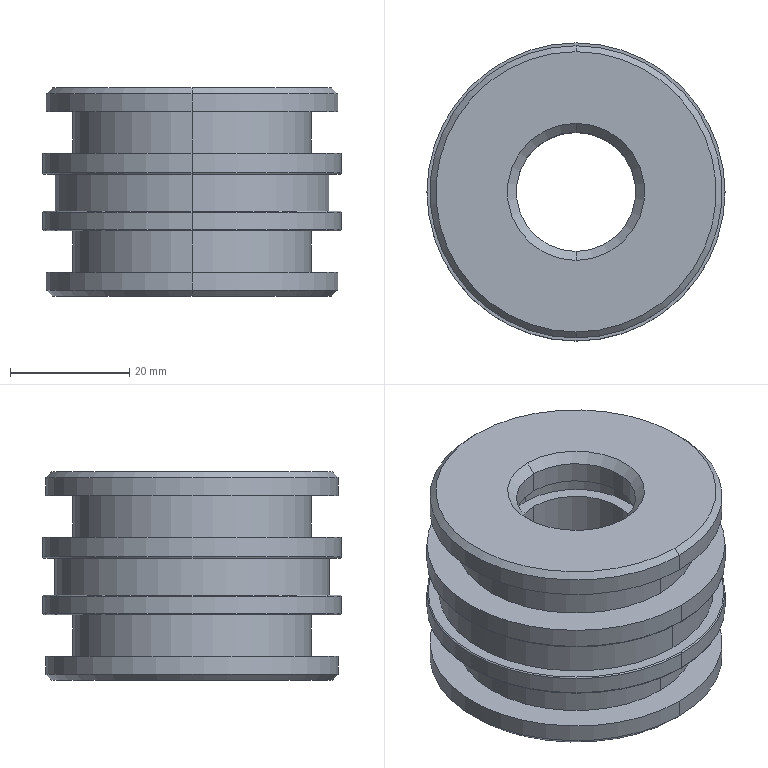Component | SolidWorks | Cylinder-1_Piston-1 | 1 solid | 42 faces | box 50 x 50 x 35 mm | volume 44660 mm3 | cylinder 20 | plane 10 | torus 6 | cone 6 | commonest cylinder face diameters 49 x4 40 x4 50 x4 20 x4 46 x2 24 x2
STEP:
#1=CARTESIAN_POINT('',(-7.109,0.06346,-12.455));
#2=VERTEX_POINT('',#1);
#3=CARTESIAN_POINT('',(-7.109,2.016,-12.455));
#4=VERTEX_POINT('',#3);
#5=CARTESIAN_POINT('',(-7.109,1.04,-12.455));
#6=DIRECTION('',(0.,-0.,-1.));
#7=DIRECTION('',(0.,1.,0.));
#8=AXIS2_PLACEMENT_3D('',#5,#6,#7);
#9=CIRCLE('',#8,0.9764);
#10=EDGE_CURVE('',#2,#4,#9,.T.);
#11=ORIENTED_EDGE('',*,*,#10,.F.);
#12=CARTESIAN_POINT('',(-7.109,0.05559,-12.447));
#13=VERTEX_POINT('',#12);
#14=CARTESIAN_POINT('',(-7.109,0.06346,-12.447));
#15=DIRECTION('',(-1.,0.,-0.));
#16=DIRECTION('',(0.,-1.,0.));
#17=AXIS2_PLACEMENT_3D('',#14,#15,#16);
#18=CIRCLE('',#17,0.007874);
#19=EDGE_CURVE('',#2,#13,#18,.T.);
#20=ORIENTED_EDGE('',*,*,#19,.T.);
#21=CARTESIAN_POINT('',(-7.109,2.024,-12.447));
#22=VERTEX_POINT('',#21);
#23=CARTESIAN_POINT('',(-7.109,1.04,-12.447));
#24=DIRECTION('',(-0.,0.,1.));
#25=DIRECTION('',(0.,1.,0.));
#26=AXIS2_PLACEMENT_3D('',#23,#24,#25);
#27=CIRCLE('',#26,0.9843);
#28=EDGE_CURVE('',#22,#13,#27,.T.);
#29=ORIENTED_EDGE('',*,*,#28,.F.);
#30=CARTESIAN_POINT('',(-7.109,2.016,-12.447));
#31=DIRECTION('',(1.,-0.,0.));
#32=DIRECTION('',(0.,1.,0.));
#33=AXIS2_PLACEMENT_3D('',#30,#31,#32);
#34=CIRCLE('',#33,0.007874);
#35=EDGE_CURVE('',#4,#22,#34,.T.);
#36=ORIENTED_EDGE('',*,*,#35,.F.);
#37=EDGE_LOOP('',(#11,#20,#29,#36));
#38=FACE_OUTER_BOUND('',#37,.T.);
#39=CARTESIAN_POINT('',(-7.109,1.04,-12.447));
#40=DIRECTION('',(-0.,0.,1.));
#41=DIRECTION('',(0.,1.,-0.));
#42=AXIS2_PLACEMENT_3D('',#39,#40,#41);
#43=TOROIDAL_SURFACE('',#42,0.9764,0.007874);
#44=ADVANCED_FACE('',(#38),#43,.T.);
#45=CARTESIAN_POINT('',(-7.109,2.016,-12.326));
#46=VERTEX_POINT('',#45);
#47=CARTESIAN_POINT('',(-7.109,0.06346,-12.326));
#48=VERTEX_POINT('',#47);
#49=CARTESIAN_POINT('',(-7.109,1.04,-12.326));
#50=DIRECTION('',(-0.,0.,1.));
#51=DIRECTION('',(0.,-1.,0.));
#52=AXIS2_PLACEMENT_3D('',#49,#50,#51);
#53=CIRCLE('',#52,0.9764);
#54=EDGE_CURVE('',#46,#48,#53,.T.);
#55=ORIENTED_EDGE('',*,*,#54,.F.);
#56=CARTESIAN_POINT('',(-7.109,2.024,-12.334));
#57=VERTEX_POINT('',#56);
#58=CARTESIAN_POINT('',(-7.109,2.016,-12.334));
#59=DIRECTION('',(-1.,-0.,-0.));
#60=DIRECTION('',(0.,-1.,0.));
#61=AXIS2_PLACEMENT_3D('',#58,#59,#60);
#62=CIRCLE('',#61,0.007874);
#63=EDGE_CURVE('',#46,#57,#62,.T.);
#64=ORIENTED_EDGE('',*,*,#63,.T.);
#65=CARTESIAN_POINT('',(-7.109,0.05559,-12.334));
#66=VERTEX_POINT('',#65);
#67=CARTESIAN_POINT('',(-7.109,1.04,-12.334));
#68=DIRECTION('',(0.,-0.,-1.));
#69=DIRECTION('',(0.,-1.,0.));
#70=AXIS2_PLACEMENT_3D('',#67,#68,#69);
#71=CIRCLE('',#70,0.9843);
#72=EDGE_CURVE('',#66,#57,#71,.T.);
#73=ORIENTED_EDGE('',*,*,#72,.F.);
#74=CARTESIAN_POINT('',(-7.109,0.06346,-12.334));
#75=DIRECTION('',(1.,-0.,0.));
#76=DIRECTION('',(0.,1.,0.));
#77=AXIS2_PLACEMENT_3D('',#74,#75,#76);
#78=CIRCLE('',#77,0.007874);
#79=EDGE_CURVE('',#48,#66,#78,.T.);
#80=ORIENTED_EDGE('',*,*,#79,.F.);
#81=EDGE_LOOP('',(#55,#64,#73,#80));
#82=FACE_OUTER_BOUND('',#81,.T.);
#83=CARTESIAN_POINT('',(-7.109,1.04,-12.334));
#84=DIRECTION('',(0.,-0.,-1.));
#85=DIRECTION('',(-0.,-1.,0.));
#86=AXIS2_PLACEMENT_3D('',#83,#84,#85);
#87=TOROIDAL_SURFACE('',#86,0.9764,0.007874);
#88=ADVANCED_FACE('',(#82),#87,.T.);
#89=CARTESIAN_POINT('',(-7.109,0.06346,-12.081));
#90=VERTEX_POINT('',#89);
#91=CARTESIAN_POINT('',(-7.109,2.016,-12.081));
#92=VERTEX_POINT('',#91);
#93=CARTESIAN_POINT('',(-7.109,1.04,-12.081));
#94=DIRECTION('',(0.,-0.,-1.));
#95=DIRECTION('',(0.,1.,0.));
#96=AXIS2_PLACEMENT_3D('',#93,#94,#95);
#97=CIRCLE('',#96,0.9764);
#98=EDGE_CURVE('',#90,#92,#97,.T.);
#99=ORIENTED_EDGE('',*,*,#98,.F.);
#100=CARTESIAN_POINT('',(-7.109,0.05559,-12.073));
#101=VERTEX_POINT('',#100);
#102=CARTESIAN_POINT('',(-7.109,0.06346,-12.073));
#103=DIRECTION('',(-1.,0.,-0.));
#104=DIRECTION('',(0.,-1.,0.));
#105=AXIS2_PLACEMENT_3D('',#102,#103,#104);
#106=CIRCLE('',#105,0.007874);
#107=EDGE_CURVE('',#90,#101,#106,.T.);
#108=ORIENTED_EDGE('',*,*,#107,.T.);
#109=CARTESIAN_POINT('',(-7.109,2.024,-12.073));
#110=VERTEX_POINT('',#109);
#111=CARTESIAN_POINT('',(-7.109,1.04,-12.073));
#112=DIRECTION('',(-0.,0.,1.));
#113=DIRECTION('',(0.,1.,0.));
#114=AXIS2_PLACEMENT_3D('',#111,#112,#113);
#115=CIRCLE('',#114,0.9843);
#116=EDGE_CURVE('',#110,#101,#115,.T.);
#117=ORIENTED_EDGE('',*,*,#116,.F.);
#118=CARTESIAN_POINT('',(-7.109,2.016,-12.073));
#119=DIRECTION('',(1.,-0.,0.));
#120=DIRECTION('',(0.,1.,0.));
#121=AXIS2_PLACEMENT_3D('',#118,#119,#120);
#122=CIRCLE('',#121,0.007874);
#123=EDGE_CURVE('',#92,#110,#122,.T.);
#124=ORIENTED_EDGE('',*,*,#123,.F.);
#125=EDGE_LOOP('',(#99,#108,#117,#124));
#126=FACE_OUTER_BOUND('',#125,.T.);
#127=CARTESIAN_POINT('',(-7.109,1.04,-12.073));
#128=DIRECTION('',(-0.,0.,1.));
#129=DIRECTION('',(0.,1.,-0.));
#130=AXIS2_PLACEMENT_3D('',#127,#128,#129);
#131=TOROIDAL_SURFACE('',#130,0.9764,0.007874);
#132=ADVANCED_FACE('',(#126),#131,.T.);
#133=CARTESIAN_POINT('',(-7.109,1.965,-11.51));
#134=VERTEX_POINT('',#133);
#135=CARTESIAN_POINT('',(-7.109,0.1146,-11.51));
#136=VERTEX_POINT('',#135);
#137=CARTESIAN_POINT('',(-7.109,1.04,-11.51));
#138=DIRECTION('',(-0.,0.,1.));
#139=DIRECTION('',(0.,-1.,0.));
#140=AXIS2_PLACEMENT_3D('',#137,#138,#139);
#141=CIRCLE('',#140,0.9252);
#142=EDGE_CURVE('',#134,#136,#141,.T.);
#143=ORIENTED_EDGE('',*,*,#142,.F.);
#144=CARTESIAN_POINT('',(-7.109,2.004,-11.549));
#145=VERTEX_POINT('',#144);
#146=CARTESIAN_POINT('',(-7.109,1.965,-11.51));
#147=DIRECTION('',(-0.,0.7071,-0.7071));
#148=VECTOR('',#147,39.37);
#149=LINE('',#146,#148);
#150=EDGE_CURVE('',#134,#145,#149,.T.);
#151=ORIENTED_EDGE('',*,*,#150,.T.);
#152=CARTESIAN_POINT('',(-7.109,0.07527,-11.549));
#153=VERTEX_POINT('',#152);
#154=CARTESIAN_POINT('',(-7.109,1.04,-11.549));
#155=DIRECTION('',(0.,-0.,-1.));
#156=DIRECTION('',(0.,-1.,0.));
#157=AXIS2_PLACEMENT_3D('',#154,#155,#156);
#158=CIRCLE('',#157,0.9646);
#159=EDGE_CURVE('',#153,#145,#158,.T.);
#160=ORIENTED_EDGE('',*,*,#159,.F.);
#161=CARTESIAN_POINT('',(-7.109,0.1146,-11.51));
#162=DIRECTION('',(-0.,-0.7071,-0.7071));
#163=VECTOR('',#162,39.37);
#164=LINE('',#161,#163);
#165=EDGE_CURVE('',#136,#153,#164,.T.);
#166=ORIENTED_EDGE('',*,*,#165,.F.);
#167=EDGE_LOOP('',(#143,#151,#160,#166));
#168=FACE_OUTER_BOUND('',#167,.T.);
#169=CARTESIAN_POINT('',(-7.109,1.04,-11.51));
#170=DIRECTION('',(0.,-0.,-1.));
#171=DIRECTION('',(0.,-1.,0.));
#172=AXIS2_PLACEMENT_3D('',#169,#170,#171);
#173=CONICAL_SURFACE('',#172,0.9252,0.7854);
#174=ADVANCED_FACE('',(#168),#173,.T.);
#175=CARTESIAN_POINT('',(-7.109,0.1146,-12.888));
#176=VERTEX_POINT('',#175);
#177=CARTESIAN_POINT('',(-7.109,1.965,-12.888));
#178=VERTEX_POINT('',#177);
#179=CARTESIAN_POINT('',(-7.109,1.04,-12.888));
#180=DIRECTION('',(0.,-0.,-1.));
#181=DIRECTION('',(0.,1.,0.));
#182=AXIS2_PLACEMENT_3D('',#179,#180,#181);
#183=CIRCLE('',#182,0.9252);
#184=EDGE_CURVE('',#176,#178,#183,.T.);
#185=ORIENTED_EDGE('',*,*,#184,.F.);
#186=CARTESIAN_POINT('',(-7.109,0.07527,-12.848));
#187=VERTEX_POINT('',#186);
#188=CARTESIAN_POINT('',(-7.109,0.07527,-12.848));
#189=DIRECTION('',(-0.,-0.7071,0.7071));
#190=VECTOR('',#189,39.37);
#191=LINE('',#188,#190);
#192=EDGE_CURVE('',#176,#187,#191,.T.);
#193=ORIENTED_EDGE('',*,*,#192,.T.);
#194=CARTESIAN_POINT('',(-7.109,2.004,-12.848));
#195=VERTEX_POINT('',#194);
#196=CARTESIAN_POINT('',(-7.109,1.04,-12.848));
#197=DIRECTION('',(-0.,0.,1.));
#198=DIRECTION('',(0.,1.,0.));
#199=AXIS2_PLACEMENT_3D('',#196,#197,#198);
#200=CIRCLE('',#199,0.9646);
#201=EDGE_CURVE('',#195,#187,#200,.T.);
#202=ORIENTED_EDGE('',*,*,#201,.F.);
#203=CARTESIAN_POINT('',(-7.109,2.004,-12.848));
#204=DIRECTION('',(0.,0.7071,0.7071));
#205=VECTOR('',#204,39.37);
#206=LINE('',#203,#205);
#207=EDGE_CURVE('',#178,#195,#206,.T.);
#208=ORIENTED_EDGE('',*,*,#207,.F.);
#209=EDGE_LOOP('',(#185,#193,#202,#208));
#210=FACE_OUTER_BOUND('',#209,.T.);
#211=CARTESIAN_POINT('',(-7.109,1.04,-12.848));
#212=DIRECTION('',(-0.,0.,1.));
#213=DIRECTION('',(0.,1.,0.));
#214=AXIS2_PLACEMENT_3D('',#211,#212,#213);
#215=CONICAL_SURFACE('',#214,0.9646,0.7854);
#216=ADVANCED_FACE('',(#210),#215,.T.);
#217=CARTESIAN_POINT('',(-7.109,0.6461,-11.569));
#218=VERTEX_POINT('',#217);
#219=CARTESIAN_POINT('',(-7.109,1.434,-11.569));
#220=VERTEX_POINT('',#219);
#221=CARTESIAN_POINT('',(-7.109,1.04,-11.569));
#222=DIRECTION('',(-0.,0.,1.));
#223=DIRECTION('',(0.,-1.,0.));
#224=AXIS2_PLACEMENT_3D('',#221,#222,#223);
#225=CIRCLE('',#224,0.3937);
#226=EDGE_CURVE('',#218,#220,#225,.T.);
#227=ORIENTED_EDGE('',*,*,#226,.F.);
#228=CARTESIAN_POINT('',(-7.109,0.5871,-11.51));
#229=VERTEX_POINT('',#228);
#230=CARTESIAN_POINT('',(-7.109,0.6461,-11.569));
#231=DIRECTION('',(-0.,-0.7071,0.7071));
#232=VECTOR('',#231,39.37);
#233=LINE('',#230,#232);
#234=EDGE_CURVE('',#218,#229,#233,.T.);
#235=ORIENTED_EDGE('',*,*,#234,.T.);
#236=CARTESIAN_POINT('',(-7.109,1.493,-11.51));
#237=VERTEX_POINT('',#236);
#238=CARTESIAN_POINT('',(-7.109,1.04,-11.51));
#239=DIRECTION('',(0.,-0.,-1.));
#240=DIRECTION('',(0.,-1.,0.));
#241=AXIS2_PLACEMENT_3D('',#238,#239,#240);
#242=CIRCLE('',#241,0.4528);
#243=EDGE_CURVE('',#237,#229,#242,.T.);
#244=ORIENTED_EDGE('',*,*,#243,.F.);
#245=CARTESIAN_POINT('',(-7.109,1.434,-11.569));
#246=DIRECTION('',(0.,0.7071,0.7071));
#247=VECTOR('',#246,39.37);
#248=LINE('',#245,#247);
#249=EDGE_CURVE('',#220,#237,#248,.T.);
#250=ORIENTED_EDGE('',*,*,#249,.F.);
#251=EDGE_LOOP('',(#227,#235,#244,#250));
#252=FACE_OUTER_BOUND('',#251,.T.);
#253=CARTESIAN_POINT('',(-7.109,1.04,-11.569));
#254=DIRECTION('',(-0.,0.,1.));
#255=DIRECTION('',(0.,1.,0.));
#256=AXIS2_PLACEMENT_3D('',#253,#254,#255);
#257=CONICAL_SURFACE('',#256,0.3937,0.7854);
#258=ADVANCED_FACE('',(#252),#257,.F.);
#259=CARTESIAN_POINT('',(-7.109,2.004,-11.667));
#260=VERTEX_POINT('',#259);
#261=CARTESIAN_POINT('',(-7.109,0.07527,-11.667));
#262=VERTEX_POINT('',#261);
#263=CARTESIAN_POINT('',(-7.109,1.04,-11.667));
#264=DIRECTION('',(-0.,0.,1.));
#265=DIRECTION('',(0.,1.,0.));
#266=AXIS2_PLACEMENT_3D('',#263,#264,#265);
#267=CIRCLE('',#266,0.9646);
#268=EDGE_CURVE('',#260,#262,#267,.T.);
#269=ORIENTED_EDGE('',*,*,#268,.T.);
#270=CARTESIAN_POINT('',(-7.109,0.07527,-9.769));
#271=DIRECTION('',(-0.,0.,1.));
#272=VECTOR('',#271,39.37);
#273=LINE('',#270,#272);
#274=EDGE_CURVE('',#262,#153,#273,.T.);
#275=ORIENTED_EDGE('',*,*,#274,.T.);
#276=ORIENTED_EDGE('',*,*,#159,.T.);
#277=CARTESIAN_POINT('',(-7.109,2.004,-9.769));
#278=DIRECTION('',(-0.,0.,1.));
#279=VECTOR('',#278,39.37);
#280=LINE('',#277,#279);
#281=EDGE_CURVE('',#260,#145,#280,.T.);
#282=ORIENTED_EDGE('',*,*,#281,.F.);
#283=EDGE_LOOP('',(#269,#275,#276,#282));
#284=FACE_OUTER_BOUND('',#283,.T.);
#285=CARTESIAN_POINT('',(-7.109,1.04,-9.769));
#286=DIRECTION('',(-0.,0.,1.));
#287=DIRECTION('',(0.,1.,0.));
#288=AXIS2_PLACEMENT_3D('',#285,#286,#287);
#289=CYLINDRICAL_SURFACE('',#288,0.9646);
#290=ADVANCED_FACE('',(#284),#289,.T.);
#291=CARTESIAN_POINT('',(-7.109,1.827,-11.943));
#292=VERTEX_POINT('',#291);
#293=CARTESIAN_POINT('',(-7.109,0.2524,-11.943));
#294=VERTEX_POINT('',#293);
#295=CARTESIAN_POINT('',(-7.109,1.04,-11.943));
#296=DIRECTION('',(-0.,0.,1.));
#297=DIRECTION('',(0.,1.,0.));
#298=AXIS2_PLACEMENT_3D('',#295,#296,#297);
#299=CIRCLE('',#298,0.7874);
#300=EDGE_CURVE('',#292,#294,#299,.T.);
#301=ORIENTED_EDGE('',*,*,#300,.T.);
#302=CARTESIAN_POINT('',(-7.109,0.2524,-11.667));
#303=VERTEX_POINT('',#302);
#304=CARTESIAN_POINT('',(-7.109,0.2524,-9.769));
#305=DIRECTION('',(-0.,0.,1.));
#306=VECTOR('',#305,39.37);
#307=LINE('',#304,#306);
#308=EDGE_CURVE('',#294,#303,#307,.T.);
#309=ORIENTED_EDGE('',*,*,#308,.T.);
#310=CARTESIAN_POINT('',(-7.109,1.827,-11.667));
#311=VERTEX_POINT('',#310);
#312=CARTESIAN_POINT('',(-7.109,1.04,-11.667));
#313=DIRECTION('',(-0.,0.,1.));
#314=DIRECTION('',(0.,1.,0.));
#315=AXIS2_PLACEMENT_3D('',#312,#313,#314);
#316=CIRCLE('',#315,0.7874);
#317=EDGE_CURVE('',#311,#303,#316,.T.);
#318=ORIENTED_EDGE('',*,*,#317,.F.);
#319=CARTESIAN_POINT('',(-7.109,1.827,-9.769));
#320=DIRECTION('',(-0.,0.,1.));
#321=VECTOR('',#320,39.37);
#322=LINE('',#319,#321);
#323=EDGE_CURVE('',#292,#311,#322,.T.);
#324=ORIENTED_EDGE('',*,*,#323,.F.);
#325=EDGE_LOOP('',(#301,#309,#318,#324));
#326=FACE_OUTER_BOUND('',#325,.T.);
#327=CARTESIAN_POINT('',(-7.109,1.04,-9.769));
#328=DIRECTION('',(-0.,0.,1.));
#329=DIRECTION('',(0.,1.,0.));
#330=AXIS2_PLACEMENT_3D('',#327,#328,#329);
#331=CYLINDRICAL_SURFACE('',#330,0.7874);
#332=ADVANCED_FACE('',(#326),#331,.T.);
#333=ORIENTED_EDGE('',*,*,#116,.T.);
#334=CARTESIAN_POINT('',(-7.109,0.05559,-11.943));
#335=VERTEX_POINT('',#334);
#336=CARTESIAN_POINT('',(-7.109,0.05559,-9.769));
#337=DIRECTION('',(-0.,0.,1.));
#338=VECTOR('',#337,39.37);
#339=LINE('',#336,#338);
#340=EDGE_CURVE('',#101,#335,#339,.T.);
#341=ORIENTED_EDGE('',*,*,#340,.T.);
#342=CARTESIAN_POINT('',(-7.109,2.024,-11.943));
#343=VERTEX_POINT('',#342);
#344=CARTESIAN_POINT('',(-7.109,1.04,-11.943));
#345=DIRECTION('',(-0.,0.,1.));
#346=DIRECTION('',(0.,1.,0.));
#347=AXIS2_PLACEMENT_3D('',#344,#345,#346);
#348=CIRCLE('',#347,0.9843);
#349=EDGE_CURVE('',#343,#335,#348,.T.);
#350=ORIENTED_EDGE('',*,*,#349,.F.);
#351=CARTESIAN_POINT('',(-7.109,2.024,-9.769));
#352=DIRECTION('',(-0.,0.,1.));
#353=VECTOR('',#352,39.37);
#354=LINE('',#351,#353);
#355=EDGE_CURVE('',#110,#343,#354,.T.);
#356=ORIENTED_EDGE('',*,*,#355,.F.);
#357=EDGE_LOOP('',(#333,#341,#350,#356));
#358=FACE_OUTER_BOUND('',#357,.T.);
#359=CARTESIAN_POINT('',(-7.109,1.04,-9.769));
#360=DIRECTION('',(-0.,0.,1.));
#361=DIRECTION('',(0.,1.,0.));
#362=AXIS2_PLACEMENT_3D('',#359,#360,#361);
#363=CYLINDRICAL_SURFACE('',#362,0.9843);
#364=ADVANCED_FACE('',(#358),#363,.T.);
#365=CARTESIAN_POINT('',(-7.109,1.945,-12.326));
#366=VERTEX_POINT('',#365);
#367=CARTESIAN_POINT('',(-7.109,0.1343,-12.326));
#368=VERTEX_POINT('',#367);
#369=CARTESIAN_POINT('',(-7.109,1.04,-12.326));
#370=DIRECTION('',(-0.,0.,1.));
#371=DIRECTION('',(0.,1.,0.));
#372=AXIS2_PLACEMENT_3D('',#369,#370,#371);
#373=CIRCLE('',#372,0.9055);
#374=EDGE_CURVE('',#366,#368,#373,.T.);
#375=ORIENTED_EDGE('',*,*,#374,.T.);
#376=CARTESIAN_POINT('',(-7.109,0.1343,-12.081));
#377=VERTEX_POINT('',#376);
#378=CARTESIAN_POINT('',(-7.109,0.1343,-9.769));
#379=DIRECTION('',(-0.,0.,1.));
#380=VECTOR('',#379,39.37);
#381=LINE('',#378,#380);
#382=EDGE_CURVE('',#368,#377,#381,.T.);
#383=ORIENTED_EDGE('',*,*,#382,.T.);
#384=CARTESIAN_POINT('',(-7.109,1.945,-12.081));
#385=VERTEX_POINT('',#384);
#386=CARTESIAN_POINT('',(-7.109,1.04,-12.081));
#387=DIRECTION('',(-0.,0.,1.));
#388=DIRECTION('',(0.,1.,0.));
#389=AXIS2_PLACEMENT_3D('',#386,#387,#388);
#390=CIRCLE('',#389,0.9055);
#391=EDGE_CURVE('',#385,#377,#390,.T.);
#392=ORIENTED_EDGE('',*,*,#391,.F.);
#393=CARTESIAN_POINT('',(-7.109,1.945,-9.769));
#394=DIRECTION('',(-0.,0.,1.));
#395=VECTOR('',#394,39.37);
#396=LINE('',#393,#395);
#397=EDGE_CURVE('',#366,#385,#396,.T.);
#398=ORIENTED_EDGE('',*,*,#397,.F.);
#399=EDGE_LOOP('',(#375,#383,#392,#398));
#400=FACE_OUTER_BOUND('',#399,.T.);
#401=CARTESIAN_POINT('',(-7.109,1.04,-9.769));
#402=DIRECTION('',(-0.,0.,1.));
#403=DIRECTION('',(0.,1.,0.));
#404=AXIS2_PLACEMENT_3D('',#401,#402,#403);
#405=CYLINDRICAL_SURFACE('',#404,0.9055);
#406=ADVANCED_FACE('',(#400),#405,.T.);
#407=ORIENTED_EDGE('',*,*,#28,.T.);
#408=CARTESIAN_POINT('',(-7.109,0.05559,-9.769));
#409=DIRECTION('',(-0.,0.,1.));
#410=VECTOR('',#409,39.37);
#411=LINE('',#408,#410);
#412=EDGE_CURVE('',#13,#66,#411,.T.);
#413=ORIENTED_EDGE('',*,*,#412,.T.);
#414=ORIENTED_EDGE('',*,*,#72,.T.);
#415=CARTESIAN_POINT('',(-7.109,2.024,-9.769));
#416=DIRECTION('',(-0.,0.,1.));
#417=VECTOR('',#416,39.37);
#418=LINE('',#415,#417);
#419=EDGE_CURVE('',#22,#57,#418,.T.);
#420=ORIENTED_EDGE('',*,*,#419,.F.);
#421=EDGE_LOOP('',(#407,#413,#414,#420));
#422=FACE_OUTER_BOUND('',#421,.T.);
#423=CARTESIAN_POINT('',(-7.109,1.04,-9.769));
#424=DIRECTION('',(-0.,0.,1.));
#425=DIRECTION('',(0.,1.,0.));
#426=AXIS2_PLACEMENT_3D('',#423,#424,#425);
#427=CYLINDRICAL_SURFACE('',#426,0.9843);
#428=ADVANCED_FACE('',(#422),#427,.T.);
#429=CARTESIAN_POINT('',(-7.109,1.827,-12.73));
#430=VERTEX_POINT('',#429);
#431=CARTESIAN_POINT('',(-7.109,0.2524,-12.73));
#432=VERTEX_POINT('',#431);
#433=CARTESIAN_POINT('',(-7.109,1.04,-12.73));
#434=DIRECTION('',(-0.,0.,1.));
#435=DIRECTION('',(0.,1.,0.));
#436=AXIS2_PLACEMENT_3D('',#433,#434,#435);
#437=CIRCLE('',#436,0.7874);
#438=EDGE_CURVE('',#430,#432,#437,.T.);
#439=ORIENTED_EDGE('',*,*,#438,.T.);
#440=CARTESIAN_POINT('',(-7.109,0.2524,-12.455));
#441=VERTEX_POINT('',#440);
#442=CARTESIAN_POINT('',(-7.109,0.2524,-9.769));
#443=DIRECTION('',(-0.,0.,1.));
#444=VECTOR('',#443,39.37);
#445=LINE('',#442,#444);
#446=EDGE_CURVE('',#432,#441,#445,.T.);
#447=ORIENTED_EDGE('',*,*,#446,.T.);
#448=CARTESIAN_POINT('',(-7.109,1.827,-12.455));
#449=VERTEX_POINT('',#448);
#450=CARTESIAN_POINT('',(-7.109,1.04,-12.455));
#451=DIRECTION('',(-0.,0.,1.));
#452=DIRECTION('',(0.,1.,0.));
#453=AXIS2_PLACEMENT_3D('',#450,#451,#452);
#454=CIRCLE('',#453,0.7874);
#455=EDGE_CURVE('',#449,#441,#454,.T.);
#456=ORIENTED_EDGE('',*,*,#455,.F.);
#457=CARTESIAN_POINT('',(-7.109,1.827,-9.769));
#458=DIRECTION('',(-0.,0.,1.));
#459=VECTOR('',#458,39.37);
#460=LINE('',#457,#459);
#461=EDGE_CURVE('',#430,#449,#460,.T.);
#462=ORIENTED_EDGE('',*,*,#461,.F.);
#463=EDGE_LOOP('',(#439,#447,#456,#462));
#464=FACE_OUTER_BOUND('',#463,.T.);
#465=CARTESIAN_POINT('',(-7.109,1.04,-9.769));
#466=DIRECTION('',(-0.,0.,1.));
#467=DIRECTION('',(0.,1.,0.));
#468=AXIS2_PLACEMENT_3D('',#465,#466,#467);
#469=CYLINDRICAL_SURFACE('',#468,0.7874);
#470=ADVANCED_FACE('',(#464),#469,.T.);
#471=ORIENTED_EDGE('',*,*,#201,.T.);
#472=CARTESIAN_POINT('',(-7.109,0.07527,-12.73));
#473=VERTEX_POINT('',#472);
#474=CARTESIAN_POINT('',(-7.109,0.07527,-9.769));
#475=DIRECTION('',(-0.,0.,1.));
#476=VECTOR('',#475,39.37);
#477=LINE('',#474,#476);
#478=EDGE_CURVE('',#187,#473,#477,.T.);
#479=ORIENTED_EDGE('',*,*,#478,.T.);
#480=CARTESIAN_POINT('',(-7.109,2.004,-12.73));
#481=VERTEX_POINT('',#480);
#482=CARTESIAN_POINT('',(-7.109,1.04,-12.73));
#483=DIRECTION('',(-0.,0.,1.));
#484=DIRECTION('',(0.,1.,0.));
#485=AXIS2_PLACEMENT_3D('',#482,#483,#484);
#486=CIRCLE('',#485,0.9646);
#487=EDGE_CURVE('',#481,#473,#486,.T.);
#488=ORIENTED_EDGE('',*,*,#487,.F.);
#489=CARTESIAN_POINT('',(-7.109,2.004,-9.769));
#490=DIRECTION('',(-0.,0.,1.));
#491=VECTOR('',#490,39.37);
#492=LINE('',#489,#491);
#493=EDGE_CURVE('',#195,#481,#492,.T.);
#494=ORIENTED_EDGE('',*,*,#493,.F.);
#495=EDGE_LOOP('',(#471,#479,#488,#494));
#496=FACE_OUTER_BOUND('',#495,.T.);
#497=CARTESIAN_POINT('',(-7.109,1.04,-9.769));
#498=DIRECTION('',(-0.,0.,1.));
#499=DIRECTION('',(0.,1.,0.));
#500=AXIS2_PLACEMENT_3D('',#497,#498,#499);
#501=CYLINDRICAL_SURFACE('',#500,0.9646);
#502=ADVANCED_FACE('',(#496),#501,.T.);
#503=CARTESIAN_POINT('',(-7.109,0.6461,-12.888));
#504=VERTEX_POINT('',#503);
#505=CARTESIAN_POINT('',(-7.109,1.434,-12.888));
#506=VERTEX_POINT('',#505);
#507=CARTESIAN_POINT('',(-7.109,1.04,-12.888));
#508=DIRECTION('',(-0.,0.,1.));
#509=DIRECTION('',(0.,1.,0.));
#510=AXIS2_PLACEMENT_3D('',#507,#508,#509);
#511=CIRCLE('',#510,0.3937);
#512=EDGE_CURVE('',#504,#506,#511,.T.);
#513=ORIENTED_EDGE('',*,*,#512,.F.);
#514=CARTESIAN_POINT('',(-7.109,0.6461,-11.833));
#515=VERTEX_POINT('',#514);
#516=CARTESIAN_POINT('',(-7.109,0.6461,-9.769));
#517=DIRECTION('',(-0.,0.,1.));
#518=VECTOR('',#517,39.37);
#519=LINE('',#516,#518);
#520=EDGE_CURVE('',#504,#515,#519,.T.);
#521=ORIENTED_EDGE('',*,*,#520,.T.);
#522=CARTESIAN_POINT('',(-7.109,1.434,-11.833));
#523=VERTEX_POINT('',#522);
#524=CARTESIAN_POINT('',(-7.109,1.04,-11.833));
#525=DIRECTION('',(-0.,0.,1.));
#526=DIRECTION('',(0.,1.,0.));
#527=AXIS2_PLACEMENT_3D('',#524,#525,#526);
#528=CIRCLE('',#527,0.3937);
#529=EDGE_CURVE('',#515,#523,#528,.T.);
#530=ORIENTED_EDGE('',*,*,#529,.T.);
#531=CARTESIAN_POINT('',(-7.109,1.434,-9.769));
#532=DIRECTION('',(-0.,0.,1.));
#533=VECTOR('',#532,39.37);
#534=LINE('',#531,#533);
#535=EDGE_CURVE('',#506,#523,#534,.T.);
#536=ORIENTED_EDGE('',*,*,#535,.F.);
#537=EDGE_LOOP('',(#513,#521,#530,#536));
#538=FACE_OUTER_BOUND('',#537,.T.);
#539=CARTESIAN_POINT('',(-7.109,1.04,-9.769));
#540=DIRECTION('',(-0.,0.,1.));
#541=DIRECTION('',(0.,1.,0.));
#542=AXIS2_PLACEMENT_3D('',#539,#540,#541);
#543=CYLINDRICAL_SURFACE('',#542,0.3937);
#544=ADVANCED_FACE('',(#538),#543,.F.);
#545=CARTESIAN_POINT('',(-7.109,0.5674,-11.833));
#546=VERTEX_POINT('',#545);
#547=CARTESIAN_POINT('',(-7.109,1.512,-11.833));
#548=VERTEX_POINT('',#547);
#549=CARTESIAN_POINT('',(-7.109,1.04,-11.833));
#550=DIRECTION('',(-0.,0.,1.));
#551=DIRECTION('',(0.,1.,0.));
#552=AXIS2_PLACEMENT_3D('',#549,#550,#551);
#553=CIRCLE('',#552,0.4724);
#554=EDGE_CURVE('',#546,#548,#553,.T.);
#555=ORIENTED_EDGE('',*,*,#554,.F.);
#556=CARTESIAN_POINT('',(-7.109,0.5674,-11.707));
#557=VERTEX_POINT('',#556);
#558=CARTESIAN_POINT('',(-7.109,0.5674,-9.769));
#559=DIRECTION('',(-0.,0.,1.));
#560=VECTOR('',#559,39.37);
#561=LINE('',#558,#560);
#562=EDGE_CURVE('',#546,#557,#561,.T.);
#563=ORIENTED_EDGE('',*,*,#562,.T.);
#564=CARTESIAN_POINT('',(-7.109,1.512,-11.707));
#565=VERTEX_POINT('',#564);
#566=CARTESIAN_POINT('',(-7.109,1.04,-11.707));
#567=DIRECTION('',(-0.,0.,1.));
#568=DIRECTION('',(0.,1.,0.));
#569=AXIS2_PLACEMENT_3D('',#566,#567,#568);
#570=CIRCLE('',#569,0.4724);
#571=EDGE_CURVE('',#557,#565,#570,.T.);
#572=ORIENTED_EDGE('',*,*,#571,.T.);
#573=CARTESIAN_POINT('',(-7.109,1.512,-9.769));
#574=DIRECTION('',(-0.,0.,1.));
#575=VECTOR('',#574,39.37);
#576=LINE('',#573,#575);
#577=EDGE_CURVE('',#548,#565,#576,.T.);
#578=ORIENTED_EDGE('',*,*,#577,.F.);
#579=EDGE_LOOP('',(#555,#563,#572,#578));
#580=FACE_OUTER_BOUND('',#579,.T.);
#581=CARTESIAN_POINT('',(-7.109,1.04,-9.769));
#582=DIRECTION('',(-0.,0.,1.));
#583=DIRECTION('',(0.,1.,0.));
#584=AXIS2_PLACEMENT_3D('',#581,#582,#583);
#585=CYLINDRICAL_SURFACE('',#584,0.4724);
#586=ADVANCED_FACE('',(#580),#585,.F.);
#587=CARTESIAN_POINT('',(-7.109,0.6461,-11.707));
#588=VERTEX_POINT('',#587);
#589=CARTESIAN_POINT('',(-7.109,1.434,-11.707));
#590=VERTEX_POINT('',#589);
#591=CARTESIAN_POINT('',(-7.109,1.04,-11.707));
#592=DIRECTION('',(-0.,0.,1.));
#593=DIRECTION('',(0.,1.,0.));
#594=AXIS2_PLACEMENT_3D('',#591,#592,#593);
#595=CIRCLE('',#594,0.3937);
#596=EDGE_CURVE('',#588,#590,#595,.T.);
#597=ORIENTED_EDGE('',*,*,#596,.F.);
#598=CARTESIAN_POINT('',(-7.109,0.6461,-9.769));
#599=DIRECTION('',(-0.,0.,1.));
#600=VECTOR('',#599,39.37);
#601=LINE('',#598,#600);
#602=EDGE_CURVE('',#588,#218,#601,.T.);
#603=ORIENTED_EDGE('',*,*,#602,.T.);
#604=ORIENTED_EDGE('',*,*,#226,.T.);
#605=CARTESIAN_POINT('',(-7.109,1.434,-9.769));
#606=DIRECTION('',(-0.,0.,1.));
#607=VECTOR('',#606,39.37);
#608=LINE('',#605,#607);
#609=EDGE_CURVE('',#590,#220,#608,.T.);
#610=ORIENTED_EDGE('',*,*,#609,.F.);
#611=EDGE_LOOP('',(#597,#603,#604,#610));
#612=FACE_OUTER_BOUND('',#611,.T.);
#613=CARTESIAN_POINT('',(-7.109,1.04,-9.769));
#614=DIRECTION('',(-0.,0.,1.));
#615=DIRECTION('',(0.,1.,0.));
#616=AXIS2_PLACEMENT_3D('',#613,#614,#615);
#617=CYLINDRICAL_SURFACE('',#616,0.3937);
#618=ADVANCED_FACE('',(#612),#617,.F.);
#619=CARTESIAN_POINT('',(-7.109,1.04,-11.51));
#620=DIRECTION('',(-0.,0.,1.));
#621=DIRECTION('',(0.,-1.,0.));
#622=AXIS2_PLACEMENT_3D('',#619,#620,#621);
#623=CIRCLE('',#622,0.9252);
#624=EDGE_CURVE('',#136,#134,#623,.T.);
#625=ORIENTED_EDGE('',*,*,#624,.T.);
#626=ORIENTED_EDGE('',*,*,#142,.T.);
#627=EDGE_LOOP('',(#625,#626));
#628=FACE_OUTER_BOUND('',#627,.T.);
#629=ORIENTED_EDGE('',*,*,#243,.T.);
#630=CARTESIAN_POINT('',(-7.109,1.04,-11.51));
#631=DIRECTION('',(0.,-0.,-1.));
#632=DIRECTION('',(0.,-1.,0.));
#633=AXIS2_PLACEMENT_3D('',#630,#631,#632);
#634=CIRCLE('',#633,0.4528);
#635=EDGE_CURVE('',#229,#237,#634,.T.);
#636=ORIENTED_EDGE('',*,*,#635,.T.);
#637=EDGE_LOOP('',(#629,#636));
#638=FACE_BOUND('',#637,.T.);
#639=CARTESIAN_POINT('',(-8.073,1.04,-11.51));
#640=DIRECTION('',(0.,-0.,-1.));
#641=DIRECTION('',(-0.,-1.,0.));
#642=AXIS2_PLACEMENT_3D('',#639,#640,#641);
#643=PLANE('',#642);
#644=ADVANCED_FACE('',(#628,#638),#643,.F.);
#645=ORIENTED_EDGE('',*,*,#602,.F.);
#646=CARTESIAN_POINT('',(-7.109,1.04,-11.707));
#647=DIRECTION('',(-0.,0.,1.));
#648=DIRECTION('',(0.,1.,0.));
#649=AXIS2_PLACEMENT_3D('',#646,#647,#648);
#650=CIRCLE('',#649,0.3937);
#651=EDGE_CURVE('',#590,#588,#650,.T.);
#652=ORIENTED_EDGE('',*,*,#651,.F.);
#653=ORIENTED_EDGE('',*,*,#609,.T.);
#654=CARTESIAN_POINT('',(-7.109,1.04,-11.569));
#655=DIRECTION('',(-0.,0.,1.));
#656=DIRECTION('',(0.,-1.,0.));
#657=AXIS2_PLACEMENT_3D('',#654,#655,#656);
#658=CIRCLE('',#657,0.3937);
#659=EDGE_CURVE('',#220,#218,#658,.T.);
#660=ORIENTED_EDGE('',*,*,#659,.T.);
#661=EDGE_LOOP('',(#645,#652,#653,#660));
#662=FACE_OUTER_BOUND('',#661,.T.);
#663=CARTESIAN_POINT('',(-7.109,1.04,-9.769));
#664=DIRECTION('',(-0.,0.,1.));
#665=DIRECTION('',(0.,1.,0.));
#666=AXIS2_PLACEMENT_3D('',#663,#664,#665);
#667=CYLINDRICAL_SURFACE('',#666,0.3937);
#668=ADVANCED_FACE('',(#662),#667,.F.);
#669=CARTESIAN_POINT('',(-7.109,1.04,-11.707));
#670=DIRECTION('',(-0.,0.,1.));
#671=DIRECTION('',(0.,1.,0.));
#672=AXIS2_PLACEMENT_3D('',#669,#670,#671);
#673=CIRCLE('',#672,0.4724);
#674=EDGE_CURVE('',#565,#557,#673,.T.);
#675=ORIENTED_EDGE('',*,*,#674,.F.);
#676=ORIENTED_EDGE('',*,*,#571,.F.);
#677=EDGE_LOOP('',(#675,#676));
#678=FACE_OUTER_BOUND('',#677,.T.);
#679=ORIENTED_EDGE('',*,*,#651,.T.);
#680=ORIENTED_EDGE('',*,*,#596,.T.);
#681=EDGE_LOOP('',(#679,#680));
#682=FACE_BOUND('',#681,.T.);
#683=CARTESIAN_POINT('',(-7.502,1.04,-11.707));
#684=DIRECTION('',(-0.,0.,1.));
#685=DIRECTION('',(0.,1.,-0.));
#686=AXIS2_PLACEMENT_3D('',#683,#684,#685);
#687=PLANE('',#686);
#688=ADVANCED_FACE('',(#678,#682),#687,.F.);
#689=ORIENTED_EDGE('',*,*,#562,.F.);
#690=CARTESIAN_POINT('',(-7.109,1.04,-11.833));
#691=DIRECTION('',(-0.,0.,1.));
#692=DIRECTION('',(0.,1.,0.));
#693=AXIS2_PLACEMENT_3D('',#690,#691,#692);
#694=CIRCLE('',#693,0.4724);
#695=EDGE_CURVE('',#548,#546,#694,.T.);
#696=ORIENTED_EDGE('',*,*,#695,.F.);
#697=ORIENTED_EDGE('',*,*,#577,.T.);
#698=ORIENTED_EDGE('',*,*,#674,.T.);
#699=EDGE_LOOP('',(#689,#696,#697,#698));
#700=FACE_OUTER_BOUND('',#699,.T.);
#701=CARTESIAN_POINT('',(-7.109,1.04,-9.769));
#702=DIRECTION('',(-0.,0.,1.));
#703=DIRECTION('',(0.,1.,0.));
#704=AXIS2_PLACEMENT_3D('',#701,#702,#703);
#705=CYLINDRICAL_SURFACE('',#704,0.4724);
#706=ADVANCED_FACE('',(#700),#705,.F.);
#707=CARTESIAN_POINT('',(-7.109,1.04,-11.833));
#708=DIRECTION('',(-0.,0.,1.));
#709=DIRECTION('',(0.,1.,0.));
#710=AXIS2_PLACEMENT_3D('',#707,#708,#709);
#711=CIRCLE('',#710,0.3937);
#712=EDGE_CURVE('',#523,#515,#711,.T.);
#713=ORIENTED_EDGE('',*,*,#712,.F.);
#714=ORIENTED_EDGE('',*,*,#529,.F.);
#715=EDGE_LOOP('',(#713,#714));
#716=FACE_BOUND('',#715,.T.);
#717=ORIENTED_EDGE('',*,*,#695,.T.);
#718=ORIENTED_EDGE('',*,*,#554,.T.);
#719=EDGE_LOOP('',(#717,#718));
#720=FACE_OUTER_BOUND('',#719,.T.);
#721=CARTESIAN_POINT('',(-7.581,1.04,-11.833));
#722=DIRECTION('',(0.,-0.,-1.));
#723=DIRECTION('',(-0.,-1.,0.));
#724=AXIS2_PLACEMENT_3D('',#721,#722,#723);
#725=PLANE('',#724);
#726=ADVANCED_FACE('',(#716,#720),#725,.F.);
#727=ORIENTED_EDGE('',*,*,#520,.F.);
#728=CARTESIAN_POINT('',(-7.109,1.04,-12.888));
#729=DIRECTION('',(-0.,0.,1.));
#730=DIRECTION('',(0.,1.,0.));
#731=AXIS2_PLACEMENT_3D('',#728,#729,#730);
#732=CIRCLE('',#731,0.3937);
#733=EDGE_CURVE('',#506,#504,#732,.T.);
#734=ORIENTED_EDGE('',*,*,#733,.F.);
#735=ORIENTED_EDGE('',*,*,#535,.T.);
#736=ORIENTED_EDGE('',*,*,#712,.T.);
#737=EDGE_LOOP('',(#727,#734,#735,#736));
#738=FACE_OUTER_BOUND('',#737,.T.);
#739=CARTESIAN_POINT('',(-7.109,1.04,-9.769));
#740=DIRECTION('',(-0.,0.,1.));
#741=DIRECTION('',(0.,1.,0.));
#742=AXIS2_PLACEMENT_3D('',#739,#740,#741);
#743=CYLINDRICAL_SURFACE('',#742,0.3937);
#744=ADVANCED_FACE('',(#738),#743,.F.);
#745=CARTESIAN_POINT('',(-7.109,1.04,-12.888));
#746=DIRECTION('',(0.,-0.,-1.));
#747=DIRECTION('',(0.,1.,0.));
#748=AXIS2_PLACEMENT_3D('',#745,#746,#747);
#749=CIRCLE('',#748,0.9252);
#750=EDGE_CURVE('',#178,#176,#749,.T.);
#751=ORIENTED_EDGE('',*,*,#750,.T.);
#752=ORIENTED_EDGE('',*,*,#184,.T.);
#753=EDGE_LOOP('',(#751,#752));
#754=FACE_OUTER_BOUND('',#753,.T.);
#755=ORIENTED_EDGE('',*,*,#733,.T.);
#756=ORIENTED_EDGE('',*,*,#512,.T.);
#757=EDGE_LOOP('',(#755,#756));
#758=FACE_BOUND('',#757,.T.);
#759=CARTESIAN_POINT('',(-7.502,1.04,-12.888));
#760=DIRECTION('',(-0.,0.,1.));
#761=DIRECTION('',(0.,1.,-0.));
#762=AXIS2_PLACEMENT_3D('',#759,#760,#761);
#763=PLANE('',#762);
#764=ADVANCED_FACE('',(#754,#758),#763,.F.);
#765=ORIENTED_EDGE('',*,*,#478,.F.);
#766=CARTESIAN_POINT('',(-7.109,1.04,-12.848));
#767=DIRECTION('',(-0.,0.,1.));
#768=DIRECTION('',(0.,1.,0.));
#769=AXIS2_PLACEMENT_3D('',#766,#767,#768);
#770=CIRCLE('',#769,0.9646);
#771=EDGE_CURVE('',#187,#195,#770,.T.);
#772=ORIENTED_EDGE('',*,*,#771,.T.);
#773=ORIENTED_EDGE('',*,*,#493,.T.);
#774=CARTESIAN_POINT('',(-7.109,1.04,-12.73));
#775=DIRECTION('',(-0.,0.,1.));
#776=DIRECTION('',(0.,1.,0.));
#777=AXIS2_PLACEMENT_3D('',#774,#775,#776);
#778=CIRCLE('',#777,0.9646);
#779=EDGE_CURVE('',#473,#481,#778,.T.);
#780=ORIENTED_EDGE('',*,*,#779,.F.);
#781=EDGE_LOOP('',(#765,#772,#773,#780));
#782=FACE_OUTER_BOUND('',#781,.T.);
#783=CARTESIAN_POINT('',(-7.109,1.04,-9.769));
#784=DIRECTION('',(-0.,0.,1.));
#785=DIRECTION('',(0.,1.,0.));
#786=AXIS2_PLACEMENT_3D('',#783,#784,#785);
#787=CYLINDRICAL_SURFACE('',#786,0.9646);
#788=ADVANCED_FACE('',(#782),#787,.T.);
#789=ORIENTED_EDGE('',*,*,#438,.F.);
#790=CARTESIAN_POINT('',(-7.109,1.04,-12.73));
#791=DIRECTION('',(-0.,0.,1.));
#792=DIRECTION('',(0.,1.,0.));
#793=AXIS2_PLACEMENT_3D('',#790,#791,#792);
#794=CIRCLE('',#793,0.7874);
#795=EDGE_CURVE('',#432,#430,#794,.T.);
#796=ORIENTED_EDGE('',*,*,#795,.F.);
#797=EDGE_LOOP('',(#789,#796));
#798=FACE_BOUND('',#797,.T.);
#799=ORIENTED_EDGE('',*,*,#487,.T.);
#800=ORIENTED_EDGE('',*,*,#779,.T.);
#801=EDGE_LOOP('',(#799,#800));
#802=FACE_OUTER_BOUND('',#801,.T.);
#803=CARTESIAN_POINT('',(-8.073,1.04,-12.73));
#804=DIRECTION('',(0.,-0.,-1.));
#805=DIRECTION('',(-0.,-1.,0.));
#806=AXIS2_PLACEMENT_3D('',#803,#804,#805);
#807=PLANE('',#806);
#808=ADVANCED_FACE('',(#798,#802),#807,.F.);
#809=ORIENTED_EDGE('',*,*,#446,.F.);
#810=ORIENTED_EDGE('',*,*,#795,.T.);
#811=ORIENTED_EDGE('',*,*,#461,.T.);
#812=CARTESIAN_POINT('',(-7.109,1.04,-12.455));
#813=DIRECTION('',(-0.,0.,1.));
#814=DIRECTION('',(0.,1.,0.));
#815=AXIS2_PLACEMENT_3D('',#812,#813,#814);
#816=CIRCLE('',#815,0.7874);
#817=EDGE_CURVE('',#441,#449,#816,.T.);
#818=ORIENTED_EDGE('',*,*,#817,.F.);
#819=EDGE_LOOP('',(#809,#810,#811,#818));
#820=FACE_OUTER_BOUND('',#819,.T.);
#821=CARTESIAN_POINT('',(-7.109,1.04,-9.769));
#822=DIRECTION('',(-0.,0.,1.));
#823=DIRECTION('',(0.,1.,0.));
#824=AXIS2_PLACEMENT_3D('',#821,#822,#823);
#825=CYLINDRICAL_SURFACE('',#824,0.7874);
#826=ADVANCED_FACE('',(#820),#825,.T.);
#827=CARTESIAN_POINT('',(-7.109,1.04,-12.455));
#828=DIRECTION('',(0.,-0.,-1.));
#829=DIRECTION('',(0.,1.,0.));
#830=AXIS2_PLACEMENT_3D('',#827,#828,#829);
#831=CIRCLE('',#830,0.9764);
#832=EDGE_CURVE('',#4,#2,#831,.T.);
#833=ORIENTED_EDGE('',*,*,#832,.T.);
#834=ORIENTED_EDGE('',*,*,#10,.T.);
#835=EDGE_LOOP('',(#833,#834));
#836=FACE_OUTER_BOUND('',#835,.T.);
#837=ORIENTED_EDGE('',*,*,#455,.T.);
#838=ORIENTED_EDGE('',*,*,#817,.T.);
#839=EDGE_LOOP('',(#837,#838));
#840=FACE_BOUND('',#839,.T.);
#841=CARTESIAN_POINT('',(-7.896,1.04,-12.455));
#842=DIRECTION('',(-0.,0.,1.));
#843=DIRECTION('',(0.,1.,-0.));
#844=AXIS2_PLACEMENT_3D('',#841,#842,#843);
#845=PLANE('',#844);
#846=ADVANCED_FACE('',(#836,#840),#845,.F.);
#847=ORIENTED_EDGE('',*,*,#412,.F.);
#848=CARTESIAN_POINT('',(-7.109,1.04,-12.447));
#849=DIRECTION('',(-0.,0.,1.));
#850=DIRECTION('',(0.,1.,0.));
#851=AXIS2_PLACEMENT_3D('',#848,#849,#850);
#852=CIRCLE('',#851,0.9843);
#853=EDGE_CURVE('',#13,#22,#852,.T.);
#854=ORIENTED_EDGE('',*,*,#853,.T.);
#855=ORIENTED_EDGE('',*,*,#419,.T.);
#856=CARTESIAN_POINT('',(-7.109,1.04,-12.334));
#857=DIRECTION('',(0.,-0.,-1.));
#858=DIRECTION('',(0.,-1.,0.));
#859=AXIS2_PLACEMENT_3D('',#856,#857,#858);
#860=CIRCLE('',#859,0.9843);
#861=EDGE_CURVE('',#57,#66,#860,.T.);
#862=ORIENTED_EDGE('',*,*,#861,.T.);
#863=EDGE_LOOP('',(#847,#854,#855,#862));
#864=FACE_OUTER_BOUND('',#863,.T.);
#865=CARTESIAN_POINT('',(-7.109,1.04,-9.769));
#866=DIRECTION('',(-0.,0.,1.));
#867=DIRECTION('',(0.,1.,0.));
#868=AXIS2_PLACEMENT_3D('',#865,#866,#867);
#869=CYLINDRICAL_SURFACE('',#868,0.9843);
#870=ADVANCED_FACE('',(#864),#869,.T.);
#871=CARTESIAN_POINT('',(-7.109,1.04,-12.326));
#872=DIRECTION('',(-0.,0.,1.));
#873=DIRECTION('',(0.,-1.,0.));
#874=AXIS2_PLACEMENT_3D('',#871,#872,#873);
#875=CIRCLE('',#874,0.9764);
#876=EDGE_CURVE('',#48,#46,#875,.T.);
#877=ORIENTED_EDGE('',*,*,#876,.T.);
#878=ORIENTED_EDGE('',*,*,#54,.T.);
#879=EDGE_LOOP('',(#877,#878));
#880=FACE_OUTER_BOUND('',#879,.T.);
#881=ORIENTED_EDGE('',*,*,#374,.F.);
#882=CARTESIAN_POINT('',(-7.109,1.04,-12.326));
#883=DIRECTION('',(-0.,0.,1.));
#884=DIRECTION('',(0.,1.,0.));
#885=AXIS2_PLACEMENT_3D('',#882,#883,#884);
#886=CIRCLE('',#885,0.9055);
#887=EDGE_CURVE('',#368,#366,#886,.T.);
#888=ORIENTED_EDGE('',*,*,#887,.F.);
#889=EDGE_LOOP('',(#881,#888));
#890=FACE_BOUND('',#889,.T.);
#891=CARTESIAN_POINT('',(-8.093,1.04,-12.326));
#892=DIRECTION('',(0.,-0.,-1.));
#893=DIRECTION('',(-0.,-1.,0.));
#894=AXIS2_PLACEMENT_3D('',#891,#892,#893);
#895=PLANE('',#894);
#896=ADVANCED_FACE('',(#880,#890),#895,.F.);
#897=ORIENTED_EDGE('',*,*,#382,.F.);
#898=ORIENTED_EDGE('',*,*,#887,.T.);
#899=ORIENTED_EDGE('',*,*,#397,.T.);
#900=CARTESIAN_POINT('',(-7.109,1.04,-12.081));
#901=DIRECTION('',(-0.,0.,1.));
#902=DIRECTION('',(0.,1.,0.));
#903=AXIS2_PLACEMENT_3D('',#900,#901,#902);
#904=CIRCLE('',#903,0.9055);
#905=EDGE_CURVE('',#377,#385,#904,.T.);
#906=ORIENTED_EDGE('',*,*,#905,.F.);
#907=EDGE_LOOP('',(#897,#898,#899,#906));
#908=FACE_OUTER_BOUND('',#907,.T.);
#909=CARTESIAN_POINT('',(-7.109,1.04,-9.769));
#910=DIRECTION('',(-0.,0.,1.));
#911=DIRECTION('',(0.,1.,0.));
#912=AXIS2_PLACEMENT_3D('',#909,#910,#911);
#913=CYLINDRICAL_SURFACE('',#912,0.9055);
#914=ADVANCED_FACE('',(#908),#913,.T.);
#915=CARTESIAN_POINT('',(-7.109,1.04,-12.081));
#916=DIRECTION('',(0.,-0.,-1.));
#917=DIRECTION('',(0.,1.,0.));
#918=AXIS2_PLACEMENT_3D('',#915,#916,#917);
#919=CIRCLE('',#918,0.9764);
#920=EDGE_CURVE('',#92,#90,#919,.T.);
#921=ORIENTED_EDGE('',*,*,#920,.T.);
#922=ORIENTED_EDGE('',*,*,#98,.T.);
#923=EDGE_LOOP('',(#921,#922));
#924=FACE_OUTER_BOUND('',#923,.T.);
#925=ORIENTED_EDGE('',*,*,#391,.T.);
#926=ORIENTED_EDGE('',*,*,#905,.T.);
#927=EDGE_LOOP('',(#925,#926));
#928=FACE_BOUND('',#927,.T.);
#929=CARTESIAN_POINT('',(-8.014,1.04,-12.081));
#930=DIRECTION('',(-0.,0.,1.));
#931=DIRECTION('',(0.,1.,-0.));
#932=AXIS2_PLACEMENT_3D('',#929,#930,#931);
#933=PLANE('',#932);
#934=ADVANCED_FACE('',(#924,#928),#933,.F.);
#935=ORIENTED_EDGE('',*,*,#340,.F.);
#936=CARTESIAN_POINT('',(-7.109,1.04,-12.073));
#937=DIRECTION('',(-0.,0.,1.));
#938=DIRECTION('',(0.,1.,0.));
#939=AXIS2_PLACEMENT_3D('',#936,#937,#938);
#940=CIRCLE('',#939,0.9843);
#941=EDGE_CURVE('',#101,#110,#940,.T.);
#942=ORIENTED_EDGE('',*,*,#941,.T.);
#943=ORIENTED_EDGE('',*,*,#355,.T.);
#944=CARTESIAN_POINT('',(-7.109,1.04,-11.943));
#945=DIRECTION('',(-0.,0.,1.));
#946=DIRECTION('',(0.,1.,0.));
#947=AXIS2_PLACEMENT_3D('',#944,#945,#946);
#948=CIRCLE('',#947,0.9843);
#949=EDGE_CURVE('',#335,#343,#948,.T.);
#950=ORIENTED_EDGE('',*,*,#949,.F.);
#951=EDGE_LOOP('',(#935,#942,#943,#950));
#952=FACE_OUTER_BOUND('',#951,.T.);
#953=CARTESIAN_POINT('',(-7.109,1.04,-9.769));
#954=DIRECTION('',(-0.,0.,1.));
#955=DIRECTION('',(0.,1.,0.));
#956=AXIS2_PLACEMENT_3D('',#953,#954,#955);
#957=CYLINDRICAL_SURFACE('',#956,0.9843);
#958=ADVANCED_FACE('',(#952),#957,.T.);
#959=ORIENTED_EDGE('',*,*,#300,.F.);
#960=CARTESIAN_POINT('',(-7.109,1.04,-11.943));
#961=DIRECTION('',(-0.,0.,1.));
#962=DIRECTION('',(0.,1.,0.));
#963=AXIS2_PLACEMENT_3D('',#960,#961,#962);
#964=CIRCLE('',#963,0.7874);
#965=EDGE_CURVE('',#294,#292,#964,.T.);
#966=ORIENTED_EDGE('',*,*,#965,.F.);
#967=EDGE_LOOP('',(#959,#966));
#968=FACE_BOUND('',#967,.T.);
#969=ORIENTED_EDGE('',*,*,#349,.T.);
#970=ORIENTED_EDGE('',*,*,#949,.T.);
#971=EDGE_LOOP('',(#969,#970));
#972=FACE_OUTER_BOUND('',#971,.T.);
#973=CARTESIAN_POINT('',(-8.093,1.04,-11.943));
#974=DIRECTION('',(0.,-0.,-1.));
#975=DIRECTION('',(-0.,-1.,0.));
#976=AXIS2_PLACEMENT_3D('',#973,#974,#975);
#977=PLANE('',#976);
#978=ADVANCED_FACE('',(#968,#972),#977,.F.);
#979=ORIENTED_EDGE('',*,*,#308,.F.);
#980=ORIENTED_EDGE('',*,*,#965,.T.);
#981=ORIENTED_EDGE('',*,*,#323,.T.);
#982=CARTESIAN_POINT('',(-7.109,1.04,-11.667));
#983=DIRECTION('',(-0.,0.,1.));
#984=DIRECTION('',(0.,1.,0.));
#985=AXIS2_PLACEMENT_3D('',#982,#983,#984);
#986=CIRCLE('',#985,0.7874);
#987=EDGE_CURVE('',#303,#311,#986,.T.);
#988=ORIENTED_EDGE('',*,*,#987,.F.);
#989=EDGE_LOOP('',(#979,#980,#981,#988));
#990=FACE_OUTER_BOUND('',#989,.T.);
#991=CARTESIAN_POINT('',(-7.109,1.04,-9.769));
#992=DIRECTION('',(-0.,0.,1.));
#993=DIRECTION('',(0.,1.,0.));
#994=AXIS2_PLACEMENT_3D('',#991,#992,#993);
#995=CYLINDRICAL_SURFACE('',#994,0.7874);
#996=ADVANCED_FACE('',(#990),#995,.T.);
#997=ORIENTED_EDGE('',*,*,#268,.F.);
#998=CARTESIAN_POINT('',(-7.109,1.04,-11.667));
#999=DIRECTION('',(-0.,0.,1.));
#1000=DIRECTION('',(0.,1.,0.));
#1001=AXIS2_PLACEMENT_3D('',#998,#999,#1000);
#1002=CIRCLE('',#1001,0.9646);
#1003=EDGE_CURVE('',#262,#260,#1002,.T.);
#1004=ORIENTED_EDGE('',*,*,#1003,.F.);
#1005=EDGE_LOOP('',(#997,#1004));
#1006=FACE_OUTER_BOUND('',#1005,.T.);
#1007=ORIENTED_EDGE('',*,*,#317,.T.);
#1008=ORIENTED_EDGE('',*,*,#987,.T.);
#1009=EDGE_LOOP('',(#1007,#1008));
#1010=FACE_BOUND('',#1009,.T.);
#1011=CARTESIAN_POINT('',(-7.896,1.04,-11.667));
#1012=DIRECTION('',(-0.,0.,1.));
#1013=DIRECTION('',(0.,1.,-0.));
#1014=AXIS2_PLACEMENT_3D('',#1011,#1012,#1013);
#1015=PLANE('',#1014);
#1016=ADVANCED_FACE('',(#1006,#1010),#1015,.F.);
#1017=ORIENTED_EDGE('',*,*,#274,.F.);
#1018=ORIENTED_EDGE('',*,*,#1003,.T.);
#1019=ORIENTED_EDGE('',*,*,#281,.T.);
#1020=CARTESIAN_POINT('',(-7.109,1.04,-11.549));
#1021=DIRECTION('',(0.,-0.,-1.));
#1022=DIRECTION('',(0.,-1.,0.));
#1023=AXIS2_PLACEMENT_3D('',#1020,#1021,#1022);
#1024=CIRCLE('',#1023,0.9646);
#1025=EDGE_CURVE('',#145,#153,#1024,.T.);
#1026=ORIENTED_EDGE('',*,*,#1025,.T.);
#1027=EDGE_LOOP('',(#1017,#1018,#1019,#1026));
#1028=FACE_OUTER_BOUND('',#1027,.T.);
#1029=CARTESIAN_POINT('',(-7.109,1.04,-9.769));
#1030=DIRECTION('',(-0.,0.,1.));
#1031=DIRECTION('',(0.,1.,0.));
#1032=AXIS2_PLACEMENT_3D('',#1029,#1030,#1031);
#1033=CYLINDRICAL_SURFACE('',#1032,0.9646);
#1034=ADVANCED_FACE('',(#1028),#1033,.T.);
#1035=ORIENTED_EDGE('',*,*,#234,.F.);
#1036=ORIENTED_EDGE('',*,*,#659,.F.);
#1037=ORIENTED_EDGE('',*,*,#249,.T.);
#1038=ORIENTED_EDGE('',*,*,#635,.F.);
#1039=EDGE_LOOP('',(#1035,#1036,#1037,#1038));
#1040=FACE_OUTER_BOUND('',#1039,.T.);
#1041=CARTESIAN_POINT('',(-7.109,1.04,-11.569));
#1042=DIRECTION('',(-0.,0.,1.));
#1043=DIRECTION('',(0.,1.,0.));
#1044=AXIS2_PLACEMENT_3D('',#1041,#1042,#1043);
#1045=CONICAL_SURFACE('',#1044,0.3937,0.7854);
#1046=ADVANCED_FACE('',(#1040),#1045,.F.);
#1047=ORIENTED_EDGE('',*,*,#192,.F.);
#1048=ORIENTED_EDGE('',*,*,#750,.F.);
#1049=ORIENTED_EDGE('',*,*,#207,.T.);
#1050=ORIENTED_EDGE('',*,*,#771,.F.);
#1051=EDGE_LOOP('',(#1047,#1048,#1049,#1050));
#1052=FACE_OUTER_BOUND('',#1051,.T.);
#1053=CARTESIAN_POINT('',(-7.109,1.04,-12.848));
#1054=DIRECTION('',(-0.,0.,1.));
#1055=DIRECTION('',(0.,1.,0.));
#1056=AXIS2_PLACEMENT_3D('',#1053,#1054,#1055);
#1057=CONICAL_SURFACE('',#1056,0.9646,0.7854);
#1058=ADVANCED_FACE('',(#1052),#1057,.T.);
#1059=ORIENTED_EDGE('',*,*,#150,.F.);
#1060=ORIENTED_EDGE('',*,*,#624,.F.);
#1061=ORIENTED_EDGE('',*,*,#165,.T.);
#1062=ORIENTED_EDGE('',*,*,#1025,.F.);
#1063=EDGE_LOOP('',(#1059,#1060,#1061,#1062));
#1064=FACE_OUTER_BOUND('',#1063,.T.);
#1065=CARTESIAN_POINT('',(-7.109,1.04,-11.51));
#1066=DIRECTION('',(0.,-0.,-1.));
#1067=DIRECTION('',(0.,-1.,0.));
#1068=AXIS2_PLACEMENT_3D('',#1065,#1066,#1067);
#1069=CONICAL_SURFACE('',#1068,0.9252,0.7854);
#1070=ADVANCED_FACE('',(#1064),#1069,.T.);
#1071=ORIENTED_EDGE('',*,*,#107,.F.);
#1072=ORIENTED_EDGE('',*,*,#920,.F.);
#1073=ORIENTED_EDGE('',*,*,#123,.T.);
#1074=ORIENTED_EDGE('',*,*,#941,.F.);
#1075=EDGE_LOOP('',(#1071,#1072,#1073,#1074));
#1076=FACE_OUTER_BOUND('',#1075,.T.);
#1077=CARTESIAN_POINT('',(-7.109,1.04,-12.073));
#1078=DIRECTION('',(-0.,0.,1.));
#1079=DIRECTION('',(0.,1.,-0.));
#1080=AXIS2_PLACEMENT_3D('',#1077,#1078,#1079);
#1081=TOROIDAL_SURFACE('',#1080,0.9764,0.007874);
#1082=ADVANCED_FACE('',(#1076),#1081,.T.);
#1083=ORIENTED_EDGE('',*,*,#63,.F.);
#1084=ORIENTED_EDGE('',*,*,#876,.F.);
#1085=ORIENTED_EDGE('',*,*,#79,.T.);
#1086=ORIENTED_EDGE('',*,*,#861,.F.);
#1087=EDGE_LOOP('',(#1083,#1084,#1085,#1086));
#1088=FACE_OUTER_BOUND('',#1087,.T.);
#1089=CARTESIAN_POINT('',(-7.109,1.04,-12.334));
#1090=DIRECTION('',(0.,-0.,-1.));
#1091=DIRECTION('',(-0.,-1.,0.));
#1092=AXIS2_PLACEMENT_3D('',#1089,#1090,#1091);
#1093=TOROIDAL_SURFACE('',#1092,0.9764,0.007874);
#1094=ADVANCED_FACE('',(#1088),#1093,.T.);
#1095=ORIENTED_EDGE('',*,*,#19,.F.);
#1096=ORIENTED_EDGE('',*,*,#832,.F.);
#1097=ORIENTED_EDGE('',*,*,#35,.T.);
#1098=ORIENTED_EDGE('',*,*,#853,.F.);
#1099=EDGE_LOOP('',(#1095,#1096,#1097,#1098));
#1100=FACE_OUTER_BOUND('',#1099,.T.);
#1101=CARTESIAN_POINT('',(-7.109,1.04,-12.447));
#1102=DIRECTION('',(-0.,0.,1.));
#1103=DIRECTION('',(0.,1.,-0.));
#1104=AXIS2_PLACEMENT_3D('',#1101,#1102,#1103);
#1105=TOROIDAL_SURFACE('',#1104,0.9764,0.007874);
#1106=ADVANCED_FACE('',(#1100),#1105,.T.);
#1107=CLOSED_SHELL('',(#44,#88,#132,#174,#216,#258,#290,#332,#364,#406,#428,#470,#502,#544,#586,#618,#644,#668,#688,#706,#726,#744,#764,#788,#808,#826,#846,#870,#896,#914,#934,#958,#978,#996,#1016,#1034,#1046,#1058,#1070,#1082,#1094,#1106));
#1108=MANIFOLD_SOLID_BREP('',#1107);
#1109=CARTESIAN_POINT('',(0.,0.,0.));
#1110=DIRECTION('',(0.,0.,1.));
#1111=DIRECTION('',(1.,0.,0.));
#1112=AXIS2_PLACEMENT_3D('',#1109,#1110,#1111);
#1113=(LENGTH_UNIT()NAMED_UNIT(*)SI_UNIT($,.METRE.));
#1114=LENGTH_MEASURE_WITH_UNIT(LENGTH_MEASURE(0.0254),#1113);
#1115=DIMENSIONAL_EXPONENTS(1.,0.,0.,0.,0.,0.,0.);
#1116=(CONVERSION_BASED_UNIT('',#1114)LENGTH_UNIT()NAMED_UNIT(#1115));
#1117=UNCERTAINTY_MEASURE_WITH_UNIT(LENGTH_MEASURE(0.00001),#1116,'','');
#1118=(NAMED_UNIT(*)PLANE_ANGLE_UNIT()SI_UNIT($,.RADIAN.));
#1119=(NAMED_UNIT(*)SI_UNIT($,.STERADIAN.)SOLID_ANGLE_UNIT());
#1120=(GEOMETRIC_REPRESENTATION_CONTEXT(3)GLOBAL_UNCERTAINTY_ASSIGNED_CONTEXT((#1117))GLOBAL_UNIT_ASSIGNED_CONTEXT((#1116,#1118,#1119))REPRESENTATION_CONTEXT('',''));
#1121=ADVANCED_BREP_SHAPE_REPRESENTATION('',(#1108,#1112),#1120);
#1122=COLOUR_RGB('',0.7922,0.8196,0.9333);
#1123=FILL_AREA_STYLE_COLOUR('',#1122);
#1124=FILL_AREA_STYLE('',(#1123));
#1125=SURFACE_STYLE_FILL_AREA(#1124);
#1126=SURFACE_SIDE_STYLE('',(#1125));
#1127=SURFACE_STYLE_USAGE(.BOTH.,#1126);
#1128=PRESENTATION_STYLE_ASSIGNMENT((#1127));
#1129=STYLED_ITEM('',(#1128),#1108);
#1130=(LENGTH_UNIT()NAMED_UNIT(*)SI_UNIT($,.METRE.));
#1131=LENGTH_MEASURE_WITH_UNIT(LENGTH_MEASURE(0.0254),#1130);
#1132=DIMENSIONAL_EXPONENTS(1.,0.,0.,0.,0.,0.,0.);
#1133=(CONVERSION_BASED_UNIT('',#1131)LENGTH_UNIT()NAMED_UNIT(#1132));
#1134=UNCERTAINTY_MEASURE_WITH_UNIT(LENGTH_MEASURE(0.00001),#1133,'','');
#1135=(NAMED_UNIT(*)PLANE_ANGLE_UNIT()SI_UNIT($,.RADIAN.));
#1136=(NAMED_UNIT(*)SI_UNIT($,.STERADIAN.)SOLID_ANGLE_UNIT());
#1137=(GEOMETRIC_REPRESENTATION_CONTEXT(3)GLOBAL_UNCERTAINTY_ASSIGNED_CONTEXT((#1134))GLOBAL_UNIT_ASSIGNED_CONTEXT((#1133,#1135,#1136))REPRESENTATION_CONTEXT('',''));
#1138=MECHANICAL_DESIGN_GEOMETRIC_PRESENTATION_REPRESENTATION('',(#1129),#1137);
#1139=PRESENTATION_LAYER_ASSIGNMENT('','',(#1129));